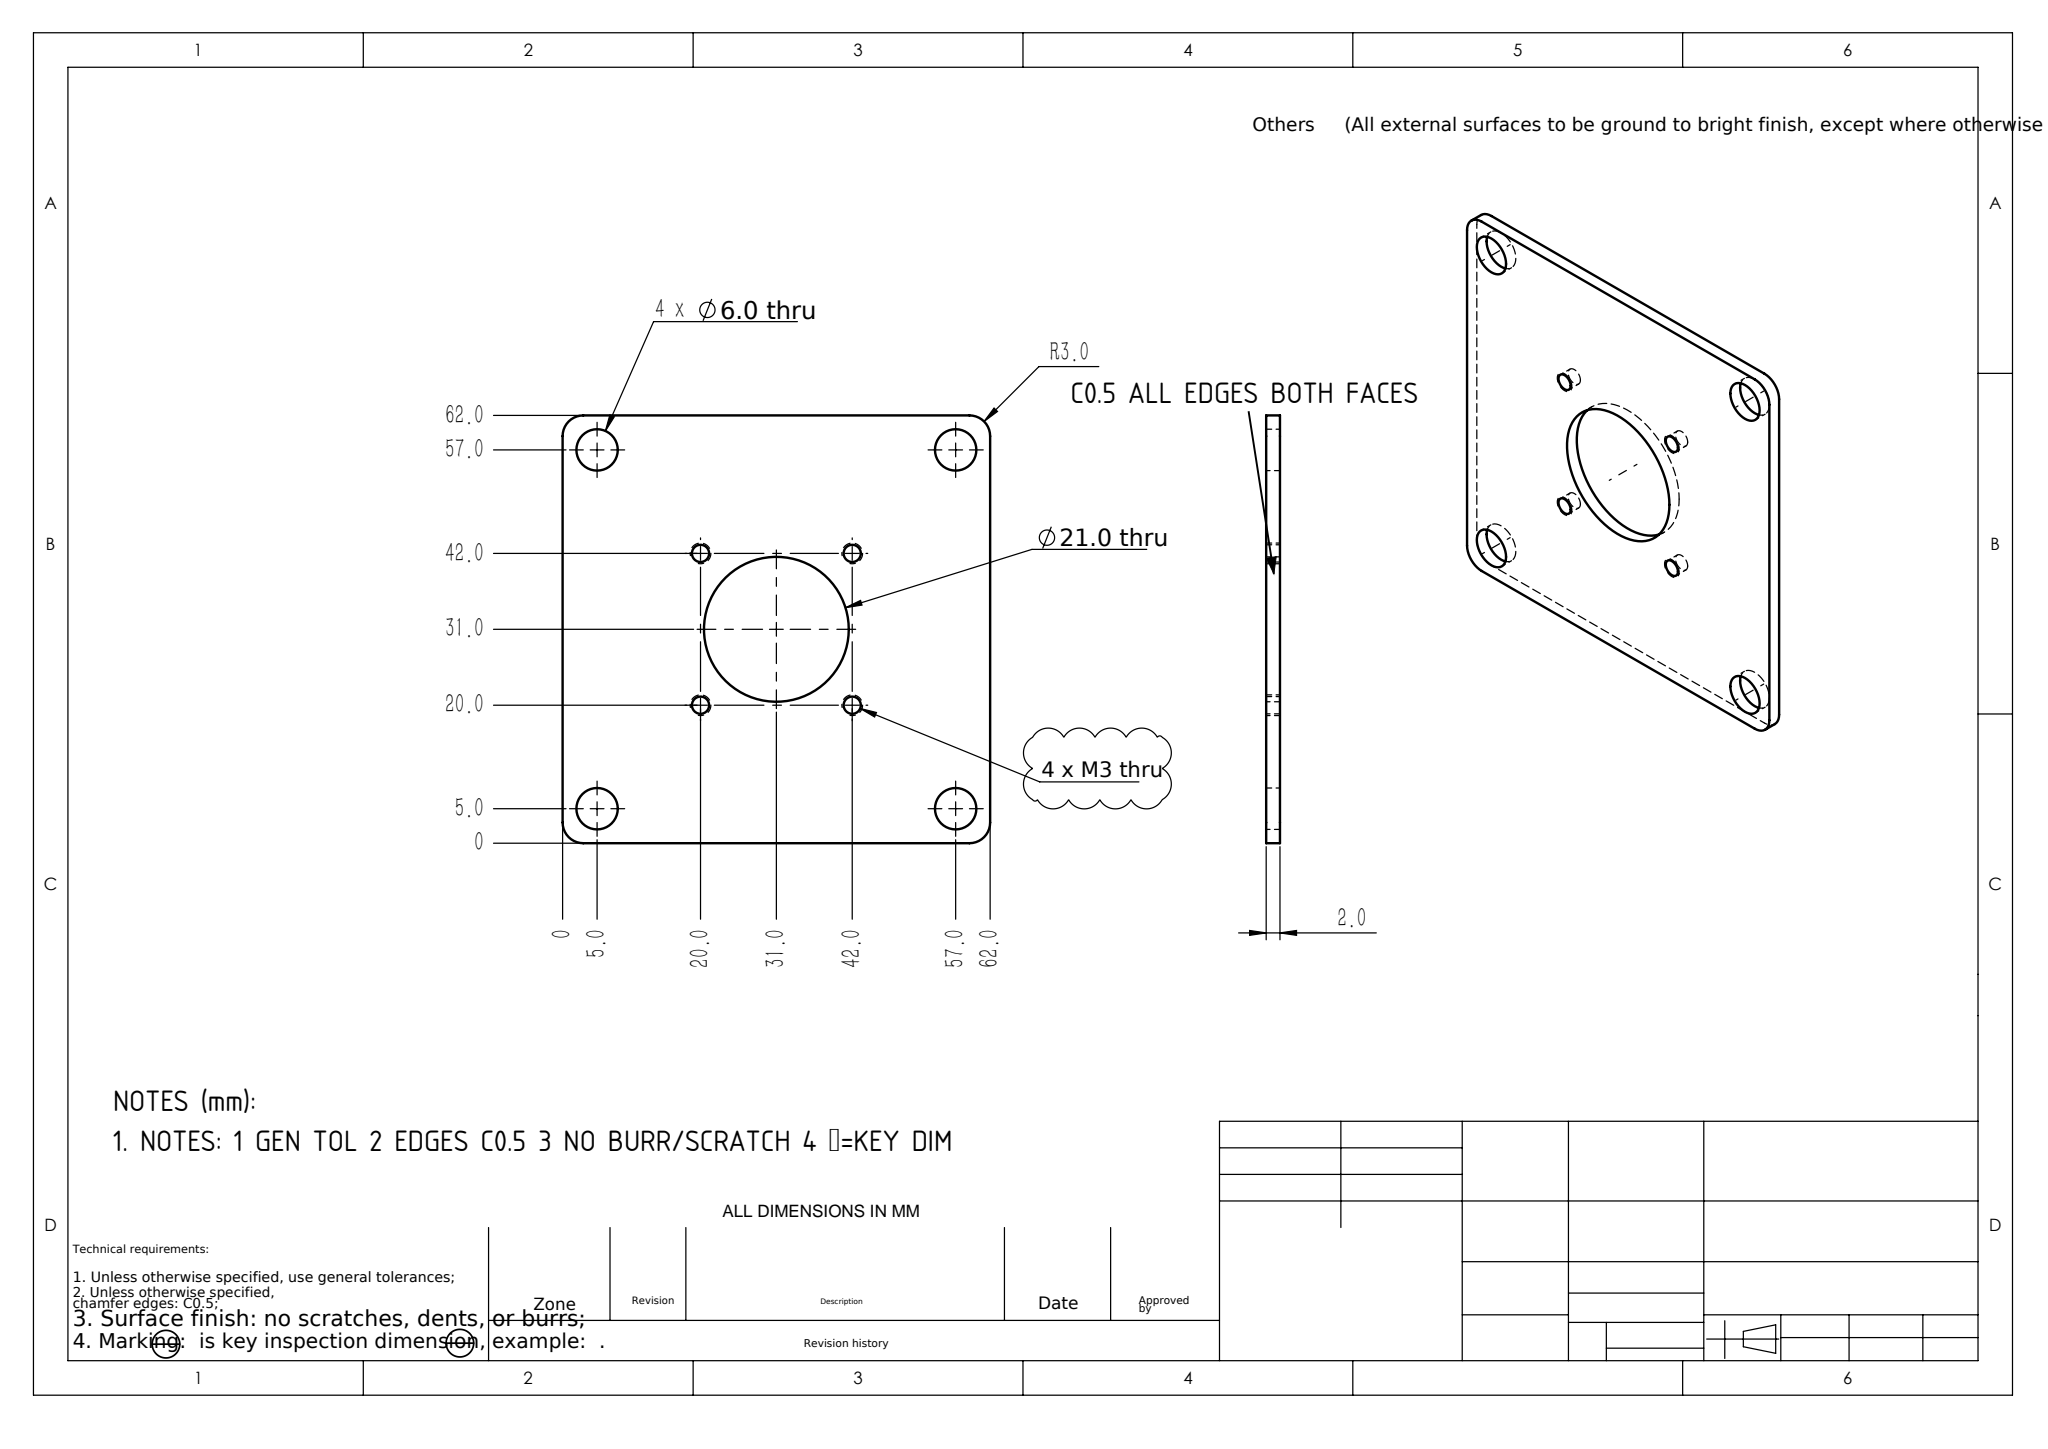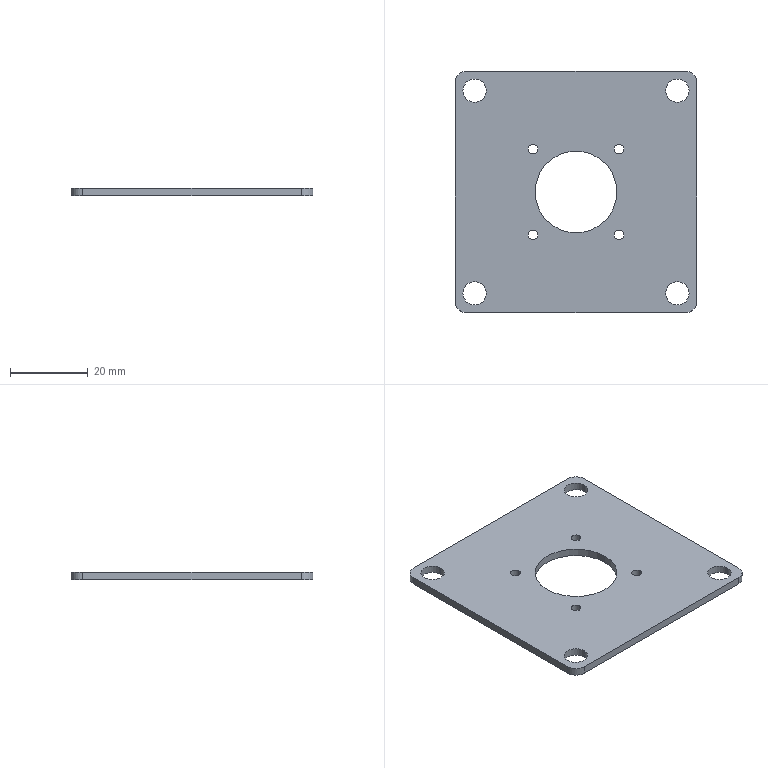Part | SolidWorks | mm | 1 solid | 28 faces | box 62 x 62 x 2 mm | volume 6714 mm3 | cylinder 22 | plane 6 | commonest cylinder face diameters 6 x12 2.5 x8 21 x2
Drawing notes:
UNLESS NOTED: BREAK ALL SHARP EDGES C0.5 (2.0 THK PLATE, BOTH FACES) | from the solid: Planes z=0.0 and z=2.0 (2.0 thk plate) with x=0/62, y=0/62 side faces; no fillet_radii or cones in STEP, so C0.5 is an unmodeled edge break
NOTES: 1 GEN TOL 2 EDGES C0.5 3 NO BURR/SCRATCH 4 Ⓒ=KEY DIM | from the solid: STEP shows plain 62.0 x 62.0 x 2.0 plate, no tol features, fillet_radii empty, cones empty: notes are general shop requirements only
build123d program:
from build123d import *

# Parameters (mm, degrees)
SKETCH1_W               = 62
SKETCH1_H               = 62
BOSS_EXTRUDE1_DEPTH     = 2
FILLET1_R               = 3
SKETCH2_R               = 10.5
CUT_EXTRUDE1_DEPTH      = 44.886
SKETCH3_R               = 3
CUT_EXTRUDE2_DEPTH      = 2
MIRROR2_COPY_1_SKETCH_R = 3
MIRROR2_COPY_1_DEPTH    = 2
M3_TAPPED_HOLE1_D       = 2.5


with BuildPart() as part:
    # Sketch1 → Boss-Extrude1 (new body)
    with BuildSketch(Plane.XY):
        Rectangle(SKETCH1_W, SKETCH1_H)
    extrude(amount=BOSS_EXTRUDE1_DEPTH)

    # Fillet1
    fillet1_edges = [part.edges().sort_by_distance(p)[0] for p in [
        (31, -31, 1),
        (-31, -31, 1),
        (-31, 31, 1),
        (31, 31, 1),
    ]]
    fillet(fillet1_edges, radius=FILLET1_R)

    # Sketch2 → Cut-Extrude1 (cut, through all)
    with BuildSketch(Plane.XY.offset(2)):
        Circle(SKETCH2_R)
    extrude(amount=-CUT_EXTRUDE1_DEPTH, mode=Mode.SUBTRACT)

    # Sketch3 → Cut-Extrude2 (cut)
    with BuildSketch(Plane.XY.offset(2)):
        with Locations((-26, 26)):
            Circle(SKETCH3_R)
    cut_extrude2 = extrude(amount=-CUT_EXTRUDE2_DEPTH, mode=Mode.SUBTRACT)

    # Mirror1: Cut-Extrude2 across plane
    add(cut_extrude2.mirror(Plane.ZX), mode=Mode.SUBTRACT)

    # Mirror2: Cut-Extrude2 across plane
    add(cut_extrude2.mirror(Plane(origin=(0, 0, 0), x_dir=(0, 0, 1), z_dir=(1, 0, 0))), mode=Mode.SUBTRACT)

    # Mirror2 copy 1 sketch → Mirror2 copy 1 (cut)
    with BuildSketch(Plane(origin=(0, 0, 2), x_dir=(-1, 0, 0), z_dir=(0, 0, 1))):
        with Locations((-26, 26)):
            Circle(MIRROR2_COPY_1_SKETCH_R)
    extrude(amount=-MIRROR2_COPY_1_DEPTH, mode=Mode.SUBTRACT)

    # M3 Tapped Hole1 (through all)
    with Locations(Plane.XY.offset(2)):
        with Locations((-11, 11), (11, 11), (11, -11), (-11, -11)):
            Hole(M3_TAPPED_HOLE1_D / 2)


solid = part.part
STEP:
#1=CARTESIAN_POINT('',(-12.25,11.,0.));
#2=VERTEX_POINT('',#1);
#3=CARTESIAN_POINT('',(-9.75,11.,0.));
#4=VERTEX_POINT('',#3);
#5=CARTESIAN_POINT('',(-11.,11.,0.));
#6=DIRECTION('',(0.,0.,1.));
#7=DIRECTION('',(1.,0.,0.));
#8=AXIS2_PLACEMENT_3D('',#5,#6,#7);
#9=CIRCLE('',#8,1.25);
#10=EDGE_CURVE('',#2,#4,#9,.T.);
#11=ORIENTED_EDGE('',*,*,#10,.F.);
#12=CARTESIAN_POINT('',(-12.25,11.,2.));
#13=VERTEX_POINT('',#12);
#14=CARTESIAN_POINT('',(-12.25,11.,2.));
#15=DIRECTION('',(0.,0.,1.));
#16=VECTOR('',#15,1000.);
#17=LINE('',#14,#16);
#18=EDGE_CURVE('',#2,#13,#17,.T.);
#19=ORIENTED_EDGE('',*,*,#18,.T.);
#20=CARTESIAN_POINT('',(-9.75,11.,2.));
#21=VERTEX_POINT('',#20);
#22=CARTESIAN_POINT('',(-11.,11.,2.));
#23=DIRECTION('',(0.,0.,1.));
#24=DIRECTION('',(1.,0.,0.));
#25=AXIS2_PLACEMENT_3D('',#22,#23,#24);
#26=CIRCLE('',#25,1.25);
#27=EDGE_CURVE('',#13,#21,#26,.T.);
#28=ORIENTED_EDGE('',*,*,#27,.T.);
#29=CARTESIAN_POINT('',(-9.75,11.,2.));
#30=DIRECTION('',(0.,0.,1.));
#31=VECTOR('',#30,1000.);
#32=LINE('',#29,#31);
#33=EDGE_CURVE('',#4,#21,#32,.T.);
#34=ORIENTED_EDGE('',*,*,#33,.F.);
#35=EDGE_LOOP('',(#11,#19,#28,#34));
#36=FACE_OUTER_BOUND('',#35,.T.);
#37=CARTESIAN_POINT('',(-11.,11.,2.));
#38=DIRECTION('',(0.,0.,1.));
#39=DIRECTION('',(1.,0.,0.));
#40=AXIS2_PLACEMENT_3D('',#37,#38,#39);
#41=CYLINDRICAL_SURFACE('',#40,1.25);
#42=ADVANCED_FACE('',(#36),#41,.F.);
#43=CARTESIAN_POINT('',(9.75,11.,0.));
#44=VERTEX_POINT('',#43);
#45=CARTESIAN_POINT('',(12.25,11.,0.));
#46=VERTEX_POINT('',#45);
#47=CARTESIAN_POINT('',(11.,11.,0.));
#48=DIRECTION('',(0.,0.,1.));
#49=DIRECTION('',(1.,0.,0.));
#50=AXIS2_PLACEMENT_3D('',#47,#48,#49);
#51=CIRCLE('',#50,1.25);
#52=EDGE_CURVE('',#44,#46,#51,.T.);
#53=ORIENTED_EDGE('',*,*,#52,.F.);
#54=CARTESIAN_POINT('',(9.75,11.,2.));
#55=VERTEX_POINT('',#54);
#56=CARTESIAN_POINT('',(9.75,11.,2.));
#57=DIRECTION('',(0.,0.,1.));
#58=VECTOR('',#57,1000.);
#59=LINE('',#56,#58);
#60=EDGE_CURVE('',#44,#55,#59,.T.);
#61=ORIENTED_EDGE('',*,*,#60,.T.);
#62=CARTESIAN_POINT('',(12.25,11.,2.));
#63=VERTEX_POINT('',#62);
#64=CARTESIAN_POINT('',(11.,11.,2.));
#65=DIRECTION('',(0.,0.,1.));
#66=DIRECTION('',(1.,0.,0.));
#67=AXIS2_PLACEMENT_3D('',#64,#65,#66);
#68=CIRCLE('',#67,1.25);
#69=EDGE_CURVE('',#55,#63,#68,.T.);
#70=ORIENTED_EDGE('',*,*,#69,.T.);
#71=CARTESIAN_POINT('',(12.25,11.,2.));
#72=DIRECTION('',(0.,0.,1.));
#73=VECTOR('',#72,1000.);
#74=LINE('',#71,#73);
#75=EDGE_CURVE('',#46,#63,#74,.T.);
#76=ORIENTED_EDGE('',*,*,#75,.F.);
#77=EDGE_LOOP('',(#53,#61,#70,#76));
#78=FACE_OUTER_BOUND('',#77,.T.);
#79=CARTESIAN_POINT('',(11.,11.,2.));
#80=DIRECTION('',(0.,0.,1.));
#81=DIRECTION('',(1.,0.,0.));
#82=AXIS2_PLACEMENT_3D('',#79,#80,#81);
#83=CYLINDRICAL_SURFACE('',#82,1.25);
#84=ADVANCED_FACE('',(#78),#83,.F.);
#85=CARTESIAN_POINT('',(9.75,-11.,0.));
#86=VERTEX_POINT('',#85);
#87=CARTESIAN_POINT('',(12.25,-11.,0.));
#88=VERTEX_POINT('',#87);
#89=CARTESIAN_POINT('',(11.,-11.,0.));
#90=DIRECTION('',(0.,0.,1.));
#91=DIRECTION('',(1.,0.,0.));
#92=AXIS2_PLACEMENT_3D('',#89,#90,#91);
#93=CIRCLE('',#92,1.25);
#94=EDGE_CURVE('',#86,#88,#93,.T.);
#95=ORIENTED_EDGE('',*,*,#94,.F.);
#96=CARTESIAN_POINT('',(9.75,-11.,2.));
#97=VERTEX_POINT('',#96);
#98=CARTESIAN_POINT('',(9.75,-11.,2.));
#99=DIRECTION('',(0.,0.,1.));
#100=VECTOR('',#99,1000.);
#101=LINE('',#98,#100);
#102=EDGE_CURVE('',#86,#97,#101,.T.);
#103=ORIENTED_EDGE('',*,*,#102,.T.);
#104=CARTESIAN_POINT('',(12.25,-11.,2.));
#105=VERTEX_POINT('',#104);
#106=CARTESIAN_POINT('',(11.,-11.,2.));
#107=DIRECTION('',(0.,0.,1.));
#108=DIRECTION('',(1.,0.,0.));
#109=AXIS2_PLACEMENT_3D('',#106,#107,#108);
#110=CIRCLE('',#109,1.25);
#111=EDGE_CURVE('',#97,#105,#110,.T.);
#112=ORIENTED_EDGE('',*,*,#111,.T.);
#113=CARTESIAN_POINT('',(12.25,-11.,2.));
#114=DIRECTION('',(0.,0.,1.));
#115=VECTOR('',#114,1000.);
#116=LINE('',#113,#115);
#117=EDGE_CURVE('',#88,#105,#116,.T.);
#118=ORIENTED_EDGE('',*,*,#117,.F.);
#119=EDGE_LOOP('',(#95,#103,#112,#118));
#120=FACE_OUTER_BOUND('',#119,.T.);
#121=CARTESIAN_POINT('',(11.,-11.,2.));
#122=DIRECTION('',(0.,0.,1.));
#123=DIRECTION('',(1.,0.,0.));
#124=AXIS2_PLACEMENT_3D('',#121,#122,#123);
#125=CYLINDRICAL_SURFACE('',#124,1.25);
#126=ADVANCED_FACE('',(#120),#125,.F.);
#127=CARTESIAN_POINT('',(-12.25,-11.,0.));
#128=VERTEX_POINT('',#127);
#129=CARTESIAN_POINT('',(-9.75,-11.,0.));
#130=VERTEX_POINT('',#129);
#131=CARTESIAN_POINT('',(-11.,-11.,0.));
#132=DIRECTION('',(0.,0.,1.));
#133=DIRECTION('',(1.,0.,0.));
#134=AXIS2_PLACEMENT_3D('',#131,#132,#133);
#135=CIRCLE('',#134,1.25);
#136=EDGE_CURVE('',#128,#130,#135,.T.);
#137=ORIENTED_EDGE('',*,*,#136,.F.);
#138=CARTESIAN_POINT('',(-12.25,-11.,2.));
#139=VERTEX_POINT('',#138);
#140=CARTESIAN_POINT('',(-12.25,-11.,2.));
#141=DIRECTION('',(0.,0.,1.));
#142=VECTOR('',#141,1000.);
#143=LINE('',#140,#142);
#144=EDGE_CURVE('',#128,#139,#143,.T.);
#145=ORIENTED_EDGE('',*,*,#144,.T.);
#146=CARTESIAN_POINT('',(-9.75,-11.,2.));
#147=VERTEX_POINT('',#146);
#148=CARTESIAN_POINT('',(-11.,-11.,2.));
#149=DIRECTION('',(0.,0.,1.));
#150=DIRECTION('',(1.,0.,0.));
#151=AXIS2_PLACEMENT_3D('',#148,#149,#150);
#152=CIRCLE('',#151,1.25);
#153=EDGE_CURVE('',#139,#147,#152,.T.);
#154=ORIENTED_EDGE('',*,*,#153,.T.);
#155=CARTESIAN_POINT('',(-9.75,-11.,2.));
#156=DIRECTION('',(0.,0.,1.));
#157=VECTOR('',#156,1000.);
#158=LINE('',#155,#157);
#159=EDGE_CURVE('',#130,#147,#158,.T.);
#160=ORIENTED_EDGE('',*,*,#159,.F.);
#161=EDGE_LOOP('',(#137,#145,#154,#160));
#162=FACE_OUTER_BOUND('',#161,.T.);
#163=CARTESIAN_POINT('',(-11.,-11.,2.));
#164=DIRECTION('',(0.,0.,1.));
#165=DIRECTION('',(1.,0.,0.));
#166=AXIS2_PLACEMENT_3D('',#163,#164,#165);
#167=CYLINDRICAL_SURFACE('',#166,1.25);
#168=ADVANCED_FACE('',(#162),#167,.F.);
#169=CARTESIAN_POINT('',(29.,26.,0.));
#170=VERTEX_POINT('',#169);
#171=CARTESIAN_POINT('',(23.,26.,0.));
#172=VERTEX_POINT('',#171);
#173=CARTESIAN_POINT('',(26.,26.,0.));
#174=DIRECTION('',(0.,0.,-1.));
#175=DIRECTION('',(-1.,0.,0.));
#176=AXIS2_PLACEMENT_3D('',#173,#174,#175);
#177=CIRCLE('',#176,3.);
#178=EDGE_CURVE('',#170,#172,#177,.T.);
#179=ORIENTED_EDGE('',*,*,#178,.T.);
#180=CARTESIAN_POINT('',(23.,26.,2.));
#181=VERTEX_POINT('',#180);
#182=CARTESIAN_POINT('',(23.,26.,-8.485));
#183=DIRECTION('',(0.,0.,1.));
#184=VECTOR('',#183,1000.);
#185=LINE('',#182,#184);
#186=EDGE_CURVE('',#172,#181,#185,.T.);
#187=ORIENTED_EDGE('',*,*,#186,.T.);
#188=CARTESIAN_POINT('',(29.,26.,2.));
#189=VERTEX_POINT('',#188);
#190=CARTESIAN_POINT('',(26.,26.,2.));
#191=DIRECTION('',(0.,0.,-1.));
#192=DIRECTION('',(-1.,0.,0.));
#193=AXIS2_PLACEMENT_3D('',#190,#191,#192);
#194=CIRCLE('',#193,3.);
#195=EDGE_CURVE('',#189,#181,#194,.T.);
#196=ORIENTED_EDGE('',*,*,#195,.F.);
#197=CARTESIAN_POINT('',(29.,26.,-8.485));
#198=DIRECTION('',(0.,0.,1.));
#199=VECTOR('',#198,1000.);
#200=LINE('',#197,#199);
#201=EDGE_CURVE('',#170,#189,#200,.T.);
#202=ORIENTED_EDGE('',*,*,#201,.F.);
#203=EDGE_LOOP('',(#179,#187,#196,#202));
#204=FACE_OUTER_BOUND('',#203,.T.);
#205=CARTESIAN_POINT('',(26.,26.,-8.485));
#206=DIRECTION('',(0.,0.,1.));
#207=DIRECTION('',(1.,0.,0.));
#208=AXIS2_PLACEMENT_3D('',#205,#206,#207);
#209=CYLINDRICAL_SURFACE('',#208,3.);
#210=ADVANCED_FACE('',(#204),#209,.F.);
#211=CARTESIAN_POINT('',(23.,-26.,0.));
#212=VERTEX_POINT('',#211);
#213=CARTESIAN_POINT('',(29.,-26.,0.));
#214=VERTEX_POINT('',#213);
#215=CARTESIAN_POINT('',(26.,-26.,0.));
#216=DIRECTION('',(0.,0.,1.));
#217=DIRECTION('',(-1.,0.,0.));
#218=AXIS2_PLACEMENT_3D('',#215,#216,#217);
#219=CIRCLE('',#218,3.);
#220=EDGE_CURVE('',#212,#214,#219,.T.);
#221=ORIENTED_EDGE('',*,*,#220,.F.);
#222=CARTESIAN_POINT('',(23.,-26.,2.));
#223=VERTEX_POINT('',#222);
#224=CARTESIAN_POINT('',(23.,-26.,-8.485));
#225=DIRECTION('',(0.,0.,1.));
#226=VECTOR('',#225,1000.);
#227=LINE('',#224,#226);
#228=EDGE_CURVE('',#212,#223,#227,.T.);
#229=ORIENTED_EDGE('',*,*,#228,.T.);
#230=CARTESIAN_POINT('',(29.,-26.,2.));
#231=VERTEX_POINT('',#230);
#232=CARTESIAN_POINT('',(26.,-26.,2.));
#233=DIRECTION('',(0.,0.,1.));
#234=DIRECTION('',(-1.,0.,0.));
#235=AXIS2_PLACEMENT_3D('',#232,#233,#234);
#236=CIRCLE('',#235,3.);
#237=EDGE_CURVE('',#223,#231,#236,.T.);
#238=ORIENTED_EDGE('',*,*,#237,.T.);
#239=CARTESIAN_POINT('',(29.,-26.,-8.485));
#240=DIRECTION('',(0.,0.,1.));
#241=VECTOR('',#240,1000.);
#242=LINE('',#239,#241);
#243=EDGE_CURVE('',#214,#231,#242,.T.);
#244=ORIENTED_EDGE('',*,*,#243,.F.);
#245=EDGE_LOOP('',(#221,#229,#238,#244));
#246=FACE_OUTER_BOUND('',#245,.T.);
#247=CARTESIAN_POINT('',(26.,-26.,-8.485));
#248=DIRECTION('',(0.,0.,1.));
#249=DIRECTION('',(1.,0.,0.));
#250=AXIS2_PLACEMENT_3D('',#247,#248,#249);
#251=CYLINDRICAL_SURFACE('',#250,3.);
#252=ADVANCED_FACE('',(#246),#251,.F.);
#253=CARTESIAN_POINT('',(-23.,-26.,0.));
#254=VERTEX_POINT('',#253);
#255=CARTESIAN_POINT('',(-29.,-26.,0.));
#256=VERTEX_POINT('',#255);
#257=CARTESIAN_POINT('',(-26.,-26.,0.));
#258=DIRECTION('',(0.,0.,-1.));
#259=DIRECTION('',(-1.,0.,0.));
#260=AXIS2_PLACEMENT_3D('',#257,#258,#259);
#261=CIRCLE('',#260,3.);
#262=EDGE_CURVE('',#254,#256,#261,.T.);
#263=ORIENTED_EDGE('',*,*,#262,.T.);
#264=CARTESIAN_POINT('',(-29.,-26.,2.));
#265=VERTEX_POINT('',#264);
#266=CARTESIAN_POINT('',(-29.,-26.,-8.485));
#267=DIRECTION('',(0.,0.,1.));
#268=VECTOR('',#267,1000.);
#269=LINE('',#266,#268);
#270=EDGE_CURVE('',#256,#265,#269,.T.);
#271=ORIENTED_EDGE('',*,*,#270,.T.);
#272=CARTESIAN_POINT('',(-23.,-26.,2.));
#273=VERTEX_POINT('',#272);
#274=CARTESIAN_POINT('',(-26.,-26.,2.));
#275=DIRECTION('',(0.,0.,-1.));
#276=DIRECTION('',(1.,0.,0.));
#277=AXIS2_PLACEMENT_3D('',#274,#275,#276);
#278=CIRCLE('',#277,3.);
#279=EDGE_CURVE('',#273,#265,#278,.T.);
#280=ORIENTED_EDGE('',*,*,#279,.F.);
#281=CARTESIAN_POINT('',(-23.,-26.,-8.485));
#282=DIRECTION('',(0.,0.,1.));
#283=VECTOR('',#282,1000.);
#284=LINE('',#281,#283);
#285=EDGE_CURVE('',#254,#273,#284,.T.);
#286=ORIENTED_EDGE('',*,*,#285,.F.);
#287=EDGE_LOOP('',(#263,#271,#280,#286));
#288=FACE_OUTER_BOUND('',#287,.T.);
#289=CARTESIAN_POINT('',(-26.,-26.,-8.485));
#290=DIRECTION('',(0.,0.,1.));
#291=DIRECTION('',(1.,0.,0.));
#292=AXIS2_PLACEMENT_3D('',#289,#290,#291);
#293=CYLINDRICAL_SURFACE('',#292,3.);
#294=ADVANCED_FACE('',(#288),#293,.F.);
#295=CARTESIAN_POINT('',(-29.,26.,0.));
#296=VERTEX_POINT('',#295);
#297=CARTESIAN_POINT('',(-23.,26.,0.));
#298=VERTEX_POINT('',#297);
#299=CARTESIAN_POINT('',(-26.,26.,0.));
#300=DIRECTION('',(0.,0.,1.));
#301=DIRECTION('',(-1.,0.,0.));
#302=AXIS2_PLACEMENT_3D('',#299,#300,#301);
#303=CIRCLE('',#302,3.);
#304=EDGE_CURVE('',#296,#298,#303,.T.);
#305=ORIENTED_EDGE('',*,*,#304,.F.);
#306=CARTESIAN_POINT('',(-29.,26.,2.));
#307=VERTEX_POINT('',#306);
#308=CARTESIAN_POINT('',(-29.,26.,-8.485));
#309=DIRECTION('',(0.,0.,1.));
#310=VECTOR('',#309,1000.);
#311=LINE('',#308,#310);
#312=EDGE_CURVE('',#296,#307,#311,.T.);
#313=ORIENTED_EDGE('',*,*,#312,.T.);
#314=CARTESIAN_POINT('',(-23.,26.,2.));
#315=VERTEX_POINT('',#314);
#316=CARTESIAN_POINT('',(-26.,26.,2.));
#317=DIRECTION('',(0.,0.,1.));
#318=DIRECTION('',(1.,0.,0.));
#319=AXIS2_PLACEMENT_3D('',#316,#317,#318);
#320=CIRCLE('',#319,3.);
#321=EDGE_CURVE('',#307,#315,#320,.T.);
#322=ORIENTED_EDGE('',*,*,#321,.T.);
#323=CARTESIAN_POINT('',(-23.,26.,-8.485));
#324=DIRECTION('',(0.,0.,1.));
#325=VECTOR('',#324,1000.);
#326=LINE('',#323,#325);
#327=EDGE_CURVE('',#298,#315,#326,.T.);
#328=ORIENTED_EDGE('',*,*,#327,.F.);
#329=EDGE_LOOP('',(#305,#313,#322,#328));
#330=FACE_OUTER_BOUND('',#329,.T.);
#331=CARTESIAN_POINT('',(-26.,26.,-8.485));
#332=DIRECTION('',(0.,0.,1.));
#333=DIRECTION('',(1.,0.,0.));
#334=AXIS2_PLACEMENT_3D('',#331,#332,#333);
#335=CYLINDRICAL_SURFACE('',#334,3.);
#336=ADVANCED_FACE('',(#330),#335,.F.);
#337=CARTESIAN_POINT('',(-10.5,0.,0.));
#338=VERTEX_POINT('',#337);
#339=CARTESIAN_POINT('',(10.5,0.,0.));
#340=VERTEX_POINT('',#339);
#341=CARTESIAN_POINT('',(0.,0.,0.));
#342=DIRECTION('',(0.,0.,1.));
#343=DIRECTION('',(1.,0.,0.));
#344=AXIS2_PLACEMENT_3D('',#341,#342,#343);
#345=CIRCLE('',#344,10.5);
#346=EDGE_CURVE('',#338,#340,#345,.T.);
#347=ORIENTED_EDGE('',*,*,#346,.F.);
#348=CARTESIAN_POINT('',(-10.5,0.,2.));
#349=VERTEX_POINT('',#348);
#350=CARTESIAN_POINT('',(-10.5,0.,0.));
#351=DIRECTION('',(0.,0.,1.));
#352=VECTOR('',#351,1000.);
#353=LINE('',#350,#352);
#354=EDGE_CURVE('',#338,#349,#353,.T.);
#355=ORIENTED_EDGE('',*,*,#354,.T.);
#356=CARTESIAN_POINT('',(10.5,0.,2.));
#357=VERTEX_POINT('',#356);
#358=CARTESIAN_POINT('',(0.,0.,2.));
#359=DIRECTION('',(0.,0.,1.));
#360=DIRECTION('',(1.,0.,0.));
#361=AXIS2_PLACEMENT_3D('',#358,#359,#360);
#362=CIRCLE('',#361,10.5);
#363=EDGE_CURVE('',#349,#357,#362,.T.);
#364=ORIENTED_EDGE('',*,*,#363,.T.);
#365=CARTESIAN_POINT('',(10.5,0.,0.));
#366=DIRECTION('',(0.,0.,1.));
#367=VECTOR('',#366,1000.);
#368=LINE('',#365,#367);
#369=EDGE_CURVE('',#340,#357,#368,.T.);
#370=ORIENTED_EDGE('',*,*,#369,.F.);
#371=EDGE_LOOP('',(#347,#355,#364,#370));
#372=FACE_OUTER_BOUND('',#371,.T.);
#373=CARTESIAN_POINT('',(0.,0.,0.));
#374=DIRECTION('',(0.,0.,1.));
#375=DIRECTION('',(1.,0.,0.));
#376=AXIS2_PLACEMENT_3D('',#373,#374,#375);
#377=CYLINDRICAL_SURFACE('',#376,10.5);
#378=ADVANCED_FACE('',(#372),#377,.F.);
#379=CARTESIAN_POINT('',(-11.,11.,0.));
#380=DIRECTION('',(0.,0.,1.));
#381=DIRECTION('',(1.,0.,0.));
#382=AXIS2_PLACEMENT_3D('',#379,#380,#381);
#383=CIRCLE('',#382,1.25);
#384=EDGE_CURVE('',#4,#2,#383,.T.);
#385=ORIENTED_EDGE('',*,*,#384,.T.);
#386=ORIENTED_EDGE('',*,*,#10,.T.);
#387=EDGE_LOOP('',(#385,#386));
#388=FACE_BOUND('',#387,.T.);
#389=CARTESIAN_POINT('',(11.,11.,0.));
#390=DIRECTION('',(0.,0.,1.));
#391=DIRECTION('',(1.,0.,0.));
#392=AXIS2_PLACEMENT_3D('',#389,#390,#391);
#393=CIRCLE('',#392,1.25);
#394=EDGE_CURVE('',#46,#44,#393,.T.);
#395=ORIENTED_EDGE('',*,*,#394,.T.);
#396=ORIENTED_EDGE('',*,*,#52,.T.);
#397=EDGE_LOOP('',(#395,#396));
#398=FACE_BOUND('',#397,.T.);
#399=CARTESIAN_POINT('',(11.,-11.,0.));
#400=DIRECTION('',(0.,0.,1.));
#401=DIRECTION('',(1.,0.,0.));
#402=AXIS2_PLACEMENT_3D('',#399,#400,#401);
#403=CIRCLE('',#402,1.25);
#404=EDGE_CURVE('',#88,#86,#403,.T.);
#405=ORIENTED_EDGE('',*,*,#404,.T.);
#406=ORIENTED_EDGE('',*,*,#94,.T.);
#407=EDGE_LOOP('',(#405,#406));
#408=FACE_BOUND('',#407,.T.);
#409=CARTESIAN_POINT('',(31.,-28.,0.));
#410=VERTEX_POINT('',#409);
#411=CARTESIAN_POINT('',(31.,28.,0.));
#412=VERTEX_POINT('',#411);
#413=CARTESIAN_POINT('',(31.,-31.,0.));
#414=DIRECTION('',(0.,1.,0.));
#415=VECTOR('',#414,1000.);
#416=LINE('',#413,#415);
#417=EDGE_CURVE('',#410,#412,#416,.T.);
#418=ORIENTED_EDGE('',*,*,#417,.F.);
#419=CARTESIAN_POINT('',(28.,-31.,0.));
#420=VERTEX_POINT('',#419);
#421=CARTESIAN_POINT('',(28.,-28.,0.));
#422=DIRECTION('',(0.,0.,-1.));
#423=DIRECTION('',(-1.,0.,0.));
#424=AXIS2_PLACEMENT_3D('',#421,#422,#423);
#425=CIRCLE('',#424,3.);
#426=EDGE_CURVE('',#410,#420,#425,.T.);
#427=ORIENTED_EDGE('',*,*,#426,.T.);
#428=CARTESIAN_POINT('',(-28.,-31.,0.));
#429=VERTEX_POINT('',#428);
#430=CARTESIAN_POINT('',(-31.,-31.,0.));
#431=DIRECTION('',(1.,0.,0.));
#432=VECTOR('',#431,1000.);
#433=LINE('',#430,#432);
#434=EDGE_CURVE('',#429,#420,#433,.T.);
#435=ORIENTED_EDGE('',*,*,#434,.F.);
#436=CARTESIAN_POINT('',(-31.,-28.,0.));
#437=VERTEX_POINT('',#436);
#438=CARTESIAN_POINT('',(-28.,-28.,0.));
#439=DIRECTION('',(0.,0.,-1.));
#440=DIRECTION('',(-1.,0.,0.));
#441=AXIS2_PLACEMENT_3D('',#438,#439,#440);
#442=CIRCLE('',#441,3.);
#443=EDGE_CURVE('',#429,#437,#442,.T.);
#444=ORIENTED_EDGE('',*,*,#443,.T.);
#445=CARTESIAN_POINT('',(-31.,28.,0.));
#446=VERTEX_POINT('',#445);
#447=CARTESIAN_POINT('',(-31.,-31.,0.));
#448=DIRECTION('',(0.,-1.,0.));
#449=VECTOR('',#448,1000.);
#450=LINE('',#447,#449);
#451=EDGE_CURVE('',#446,#437,#450,.T.);
#452=ORIENTED_EDGE('',*,*,#451,.F.);
#453=CARTESIAN_POINT('',(-28.,31.,0.));
#454=VERTEX_POINT('',#453);
#455=CARTESIAN_POINT('',(-28.,28.,0.));
#456=DIRECTION('',(0.,0.,-1.));
#457=DIRECTION('',(-1.,0.,0.));
#458=AXIS2_PLACEMENT_3D('',#455,#456,#457);
#459=CIRCLE('',#458,3.);
#460=EDGE_CURVE('',#446,#454,#459,.T.);
#461=ORIENTED_EDGE('',*,*,#460,.T.);
#462=CARTESIAN_POINT('',(28.,31.,0.));
#463=VERTEX_POINT('',#462);
#464=CARTESIAN_POINT('',(-31.,31.,0.));
#465=DIRECTION('',(-1.,0.,0.));
#466=VECTOR('',#465,1000.);
#467=LINE('',#464,#466);
#468=EDGE_CURVE('',#463,#454,#467,.T.);
#469=ORIENTED_EDGE('',*,*,#468,.F.);
#470=CARTESIAN_POINT('',(28.,28.,0.));
#471=DIRECTION('',(0.,0.,-1.));
#472=DIRECTION('',(-1.,0.,0.));
#473=AXIS2_PLACEMENT_3D('',#470,#471,#472);
#474=CIRCLE('',#473,3.);
#475=EDGE_CURVE('',#463,#412,#474,.T.);
#476=ORIENTED_EDGE('',*,*,#475,.T.);
#477=EDGE_LOOP('',(#418,#427,#435,#444,#452,#461,#469,#476));
#478=FACE_OUTER_BOUND('',#477,.T.);
#479=CARTESIAN_POINT('',(0.,0.,0.));
#480=DIRECTION('',(0.,0.,1.));
#481=DIRECTION('',(1.,0.,0.));
#482=AXIS2_PLACEMENT_3D('',#479,#480,#481);
#483=CIRCLE('',#482,10.5);
#484=EDGE_CURVE('',#340,#338,#483,.T.);
#485=ORIENTED_EDGE('',*,*,#484,.T.);
#486=ORIENTED_EDGE('',*,*,#346,.T.);
#487=EDGE_LOOP('',(#485,#486));
#488=FACE_BOUND('',#487,.T.);
#489=CARTESIAN_POINT('',(-26.,26.,0.));
#490=DIRECTION('',(0.,0.,1.));
#491=DIRECTION('',(-1.,0.,0.));
#492=AXIS2_PLACEMENT_3D('',#489,#490,#491);
#493=CIRCLE('',#492,3.);
#494=EDGE_CURVE('',#298,#296,#493,.T.);
#495=ORIENTED_EDGE('',*,*,#494,.T.);
#496=ORIENTED_EDGE('',*,*,#304,.T.);
#497=EDGE_LOOP('',(#495,#496));
#498=FACE_BOUND('',#497,.T.);
#499=ORIENTED_EDGE('',*,*,#262,.F.);
#500=CARTESIAN_POINT('',(-26.,-26.,0.));
#501=DIRECTION('',(0.,0.,-1.));
#502=DIRECTION('',(-1.,0.,0.));
#503=AXIS2_PLACEMENT_3D('',#500,#501,#502);
#504=CIRCLE('',#503,3.);
#505=EDGE_CURVE('',#256,#254,#504,.T.);
#506=ORIENTED_EDGE('',*,*,#505,.F.);
#507=EDGE_LOOP('',(#499,#506));
#508=FACE_BOUND('',#507,.T.);
#509=CARTESIAN_POINT('',(26.,-26.,0.));
#510=DIRECTION('',(0.,0.,1.));
#511=DIRECTION('',(-1.,0.,0.));
#512=AXIS2_PLACEMENT_3D('',#509,#510,#511);
#513=CIRCLE('',#512,3.);
#514=EDGE_CURVE('',#214,#212,#513,.T.);
#515=ORIENTED_EDGE('',*,*,#514,.T.);
#516=ORIENTED_EDGE('',*,*,#220,.T.);
#517=EDGE_LOOP('',(#515,#516));
#518=FACE_BOUND('',#517,.T.);
#519=ORIENTED_EDGE('',*,*,#178,.F.);
#520=CARTESIAN_POINT('',(26.,26.,0.));
#521=DIRECTION('',(0.,0.,-1.));
#522=DIRECTION('',(-1.,0.,0.));
#523=AXIS2_PLACEMENT_3D('',#520,#521,#522);
#524=CIRCLE('',#523,3.);
#525=EDGE_CURVE('',#172,#170,#524,.T.);
#526=ORIENTED_EDGE('',*,*,#525,.F.);
#527=EDGE_LOOP('',(#519,#526));
#528=FACE_BOUND('',#527,.T.);
#529=CARTESIAN_POINT('',(-11.,-11.,0.));
#530=DIRECTION('',(0.,0.,1.));
#531=DIRECTION('',(1.,0.,0.));
#532=AXIS2_PLACEMENT_3D('',#529,#530,#531);
#533=CIRCLE('',#532,1.25);
#534=EDGE_CURVE('',#130,#128,#533,.T.);
#535=ORIENTED_EDGE('',*,*,#534,.T.);
#536=ORIENTED_EDGE('',*,*,#136,.T.);
#537=EDGE_LOOP('',(#535,#536));
#538=FACE_BOUND('',#537,.T.);
#539=CARTESIAN_POINT('',(0.,0.,0.));
#540=DIRECTION('',(0.,0.,-1.));
#541=DIRECTION('',(-1.,0.,0.));
#542=AXIS2_PLACEMENT_3D('',#539,#540,#541);
#543=PLANE('',#542);
#544=ADVANCED_FACE('',(#388,#398,#408,#478,#488,#498,#508,#518,#528,#538),#543,.T.);
#545=CARTESIAN_POINT('',(31.,-28.,2.));
#546=VERTEX_POINT('',#545);
#547=CARTESIAN_POINT('',(31.,28.,2.));
#548=VERTEX_POINT('',#547);
#549=CARTESIAN_POINT('',(31.,-31.,2.));
#550=DIRECTION('',(0.,1.,0.));
#551=VECTOR('',#550,1000.);
#552=LINE('',#549,#551);
#553=EDGE_CURVE('',#546,#548,#552,.T.);
#554=ORIENTED_EDGE('',*,*,#553,.F.);
#555=CARTESIAN_POINT('',(31.,-28.,2.));
#556=DIRECTION('',(0.,0.,-1.));
#557=VECTOR('',#556,1000.);
#558=LINE('',#555,#557);
#559=EDGE_CURVE('',#546,#410,#558,.T.);
#560=ORIENTED_EDGE('',*,*,#559,.T.);
#561=ORIENTED_EDGE('',*,*,#417,.T.);
#562=CARTESIAN_POINT('',(31.,28.,2.));
#563=DIRECTION('',(0.,0.,1.));
#564=VECTOR('',#563,1000.);
#565=LINE('',#562,#564);
#566=EDGE_CURVE('',#412,#548,#565,.T.);
#567=ORIENTED_EDGE('',*,*,#566,.T.);
#568=EDGE_LOOP('',(#554,#560,#561,#567));
#569=FACE_OUTER_BOUND('',#568,.T.);
#570=CARTESIAN_POINT('',(31.,-31.,2.));
#571=DIRECTION('',(-1.,0.,0.));
#572=DIRECTION('',(0.,0.,1.));
#573=AXIS2_PLACEMENT_3D('',#570,#571,#572);
#574=PLANE('',#573);
#575=ADVANCED_FACE('',(#569),#574,.F.);
#576=ORIENTED_EDGE('',*,*,#468,.T.);
#577=CARTESIAN_POINT('',(-28.,31.,2.));
#578=VERTEX_POINT('',#577);
#579=CARTESIAN_POINT('',(-28.,31.,2.));
#580=DIRECTION('',(0.,0.,1.));
#581=VECTOR('',#580,1000.);
#582=LINE('',#579,#581);
#583=EDGE_CURVE('',#454,#578,#582,.T.);
#584=ORIENTED_EDGE('',*,*,#583,.T.);
#585=CARTESIAN_POINT('',(28.,31.,2.));
#586=VERTEX_POINT('',#585);
#587=CARTESIAN_POINT('',(-31.,31.,2.));
#588=DIRECTION('',(-1.,0.,0.));
#589=VECTOR('',#588,1000.);
#590=LINE('',#587,#589);
#591=EDGE_CURVE('',#586,#578,#590,.T.);
#592=ORIENTED_EDGE('',*,*,#591,.F.);
#593=CARTESIAN_POINT('',(28.,31.,2.));
#594=DIRECTION('',(0.,0.,-1.));
#595=VECTOR('',#594,1000.);
#596=LINE('',#593,#595);
#597=EDGE_CURVE('',#586,#463,#596,.T.);
#598=ORIENTED_EDGE('',*,*,#597,.T.);
#599=EDGE_LOOP('',(#576,#584,#592,#598));
#600=FACE_OUTER_BOUND('',#599,.T.);
#601=CARTESIAN_POINT('',(-31.,31.,2.));
#602=DIRECTION('',(0.,-1.,0.));
#603=DIRECTION('',(0.,0.,-1.));
#604=AXIS2_PLACEMENT_3D('',#601,#602,#603);
#605=PLANE('',#604);
#606=ADVANCED_FACE('',(#600),#605,.F.);
#607=ORIENTED_EDGE('',*,*,#451,.T.);
#608=CARTESIAN_POINT('',(-31.,-28.,2.));
#609=VERTEX_POINT('',#608);
#610=CARTESIAN_POINT('',(-31.,-28.,2.));
#611=DIRECTION('',(0.,0.,1.));
#612=VECTOR('',#611,1000.);
#613=LINE('',#610,#612);
#614=EDGE_CURVE('',#437,#609,#613,.T.);
#615=ORIENTED_EDGE('',*,*,#614,.T.);
#616=CARTESIAN_POINT('',(-31.,28.,2.));
#617=VERTEX_POINT('',#616);
#618=CARTESIAN_POINT('',(-31.,-31.,2.));
#619=DIRECTION('',(0.,-1.,0.));
#620=VECTOR('',#619,1000.);
#621=LINE('',#618,#620);
#622=EDGE_CURVE('',#617,#609,#621,.T.);
#623=ORIENTED_EDGE('',*,*,#622,.F.);
#624=CARTESIAN_POINT('',(-31.,28.,2.));
#625=DIRECTION('',(0.,0.,-1.));
#626=VECTOR('',#625,1000.);
#627=LINE('',#624,#626);
#628=EDGE_CURVE('',#617,#446,#627,.T.);
#629=ORIENTED_EDGE('',*,*,#628,.T.);
#630=EDGE_LOOP('',(#607,#615,#623,#629));
#631=FACE_OUTER_BOUND('',#630,.T.);
#632=CARTESIAN_POINT('',(-31.,-31.,2.));
#633=DIRECTION('',(1.,0.,0.));
#634=DIRECTION('',(0.,0.,-1.));
#635=AXIS2_PLACEMENT_3D('',#632,#633,#634);
#636=PLANE('',#635);
#637=ADVANCED_FACE('',(#631),#636,.F.);
#638=ORIENTED_EDGE('',*,*,#434,.T.);
#639=CARTESIAN_POINT('',(28.,-31.,2.));
#640=VERTEX_POINT('',#639);
#641=CARTESIAN_POINT('',(28.,-31.,2.));
#642=DIRECTION('',(0.,0.,1.));
#643=VECTOR('',#642,1000.);
#644=LINE('',#641,#643);
#645=EDGE_CURVE('',#420,#640,#644,.T.);
#646=ORIENTED_EDGE('',*,*,#645,.T.);
#647=CARTESIAN_POINT('',(-28.,-31.,2.));
#648=VERTEX_POINT('',#647);
#649=CARTESIAN_POINT('',(-31.,-31.,2.));
#650=DIRECTION('',(1.,0.,0.));
#651=VECTOR('',#650,1000.);
#652=LINE('',#649,#651);
#653=EDGE_CURVE('',#648,#640,#652,.T.);
#654=ORIENTED_EDGE('',*,*,#653,.F.);
#655=CARTESIAN_POINT('',(-28.,-31.,2.));
#656=DIRECTION('',(0.,0.,-1.));
#657=VECTOR('',#656,1000.);
#658=LINE('',#655,#657);
#659=EDGE_CURVE('',#648,#429,#658,.T.);
#660=ORIENTED_EDGE('',*,*,#659,.T.);
#661=EDGE_LOOP('',(#638,#646,#654,#660));
#662=FACE_OUTER_BOUND('',#661,.T.);
#663=CARTESIAN_POINT('',(-31.,-31.,2.));
#664=DIRECTION('',(0.,1.,0.));
#665=DIRECTION('',(0.,0.,1.));
#666=AXIS2_PLACEMENT_3D('',#663,#664,#665);
#667=PLANE('',#666);
#668=ADVANCED_FACE('',(#662),#667,.F.);
#669=CARTESIAN_POINT('',(-11.,11.,2.));
#670=DIRECTION('',(0.,0.,1.));
#671=DIRECTION('',(1.,0.,0.));
#672=AXIS2_PLACEMENT_3D('',#669,#670,#671);
#673=CIRCLE('',#672,1.25);
#674=EDGE_CURVE('',#21,#13,#673,.T.);
#675=ORIENTED_EDGE('',*,*,#674,.F.);
#676=ORIENTED_EDGE('',*,*,#27,.F.);
#677=EDGE_LOOP('',(#675,#676));
#678=FACE_BOUND('',#677,.T.);
#679=CARTESIAN_POINT('',(11.,11.,2.));
#680=DIRECTION('',(0.,0.,1.));
#681=DIRECTION('',(1.,0.,0.));
#682=AXIS2_PLACEMENT_3D('',#679,#680,#681);
#683=CIRCLE('',#682,1.25);
#684=EDGE_CURVE('',#63,#55,#683,.T.);
#685=ORIENTED_EDGE('',*,*,#684,.F.);
#686=ORIENTED_EDGE('',*,*,#69,.F.);
#687=EDGE_LOOP('',(#685,#686));
#688=FACE_BOUND('',#687,.T.);
#689=CARTESIAN_POINT('',(11.,-11.,2.));
#690=DIRECTION('',(0.,0.,1.));
#691=DIRECTION('',(1.,0.,0.));
#692=AXIS2_PLACEMENT_3D('',#689,#690,#691);
#693=CIRCLE('',#692,1.25);
#694=EDGE_CURVE('',#105,#97,#693,.T.);
#695=ORIENTED_EDGE('',*,*,#694,.F.);
#696=ORIENTED_EDGE('',*,*,#111,.F.);
#697=EDGE_LOOP('',(#695,#696));
#698=FACE_BOUND('',#697,.T.);
#699=CARTESIAN_POINT('',(-11.,-11.,2.));
#700=DIRECTION('',(0.,0.,1.));
#701=DIRECTION('',(1.,0.,0.));
#702=AXIS2_PLACEMENT_3D('',#699,#700,#701);
#703=CIRCLE('',#702,1.25);
#704=EDGE_CURVE('',#147,#139,#703,.T.);
#705=ORIENTED_EDGE('',*,*,#704,.F.);
#706=ORIENTED_EDGE('',*,*,#153,.F.);
#707=EDGE_LOOP('',(#705,#706));
#708=FACE_BOUND('',#707,.T.);
#709=ORIENTED_EDGE('',*,*,#195,.T.);
#710=CARTESIAN_POINT('',(26.,26.,2.));
#711=DIRECTION('',(0.,0.,-1.));
#712=DIRECTION('',(-1.,0.,0.));
#713=AXIS2_PLACEMENT_3D('',#710,#711,#712);
#714=CIRCLE('',#713,3.);
#715=EDGE_CURVE('',#181,#189,#714,.T.);
#716=ORIENTED_EDGE('',*,*,#715,.T.);
#717=EDGE_LOOP('',(#709,#716));
#718=FACE_BOUND('',#717,.T.);
#719=CARTESIAN_POINT('',(26.,-26.,2.));
#720=DIRECTION('',(0.,0.,1.));
#721=DIRECTION('',(-1.,0.,0.));
#722=AXIS2_PLACEMENT_3D('',#719,#720,#721);
#723=CIRCLE('',#722,3.);
#724=EDGE_CURVE('',#231,#223,#723,.T.);
#725=ORIENTED_EDGE('',*,*,#724,.F.);
#726=ORIENTED_EDGE('',*,*,#237,.F.);
#727=EDGE_LOOP('',(#725,#726));
#728=FACE_BOUND('',#727,.T.);
#729=ORIENTED_EDGE('',*,*,#279,.T.);
#730=CARTESIAN_POINT('',(-26.,-26.,2.));
#731=DIRECTION('',(0.,0.,-1.));
#732=DIRECTION('',(1.,0.,0.));
#733=AXIS2_PLACEMENT_3D('',#730,#731,#732);
#734=CIRCLE('',#733,3.);
#735=EDGE_CURVE('',#265,#273,#734,.T.);
#736=ORIENTED_EDGE('',*,*,#735,.T.);
#737=EDGE_LOOP('',(#729,#736));
#738=FACE_BOUND('',#737,.T.);
#739=CARTESIAN_POINT('',(-26.,26.,2.));
#740=DIRECTION('',(0.,0.,1.));
#741=DIRECTION('',(1.,0.,0.));
#742=AXIS2_PLACEMENT_3D('',#739,#740,#741);
#743=CIRCLE('',#742,3.);
#744=EDGE_CURVE('',#315,#307,#743,.T.);
#745=ORIENTED_EDGE('',*,*,#744,.F.);
#746=ORIENTED_EDGE('',*,*,#321,.F.);
#747=EDGE_LOOP('',(#745,#746));
#748=FACE_BOUND('',#747,.T.);
#749=CARTESIAN_POINT('',(0.,0.,2.));
#750=DIRECTION('',(0.,0.,1.));
#751=DIRECTION('',(1.,0.,0.));
#752=AXIS2_PLACEMENT_3D('',#749,#750,#751);
#753=CIRCLE('',#752,10.5);
#754=EDGE_CURVE('',#357,#349,#753,.T.);
#755=ORIENTED_EDGE('',*,*,#754,.F.);
#756=ORIENTED_EDGE('',*,*,#363,.F.);
#757=EDGE_LOOP('',(#755,#756));
#758=FACE_BOUND('',#757,.T.);
#759=ORIENTED_EDGE('',*,*,#653,.T.);
#760=CARTESIAN_POINT('',(28.,-28.,2.));
#761=DIRECTION('',(0.,0.,1.));
#762=DIRECTION('',(-1.,0.,0.));
#763=AXIS2_PLACEMENT_3D('',#760,#761,#762);
#764=CIRCLE('',#763,3.);
#765=EDGE_CURVE('',#640,#546,#764,.T.);
#766=ORIENTED_EDGE('',*,*,#765,.T.);
#767=ORIENTED_EDGE('',*,*,#553,.T.);
#768=CARTESIAN_POINT('',(28.,28.,2.));
#769=DIRECTION('',(0.,0.,1.));
#770=DIRECTION('',(-1.,0.,0.));
#771=AXIS2_PLACEMENT_3D('',#768,#769,#770);
#772=CIRCLE('',#771,3.);
#773=EDGE_CURVE('',#548,#586,#772,.T.);
#774=ORIENTED_EDGE('',*,*,#773,.T.);
#775=ORIENTED_EDGE('',*,*,#591,.T.);
#776=CARTESIAN_POINT('',(-28.,28.,2.));
#777=DIRECTION('',(0.,0.,1.));
#778=DIRECTION('',(-1.,0.,0.));
#779=AXIS2_PLACEMENT_3D('',#776,#777,#778);
#780=CIRCLE('',#779,3.);
#781=EDGE_CURVE('',#578,#617,#780,.T.);
#782=ORIENTED_EDGE('',*,*,#781,.T.);
#783=ORIENTED_EDGE('',*,*,#622,.T.);
#784=CARTESIAN_POINT('',(-28.,-28.,2.));
#785=DIRECTION('',(0.,0.,1.));
#786=DIRECTION('',(-1.,0.,0.));
#787=AXIS2_PLACEMENT_3D('',#784,#785,#786);
#788=CIRCLE('',#787,3.);
#789=EDGE_CURVE('',#609,#648,#788,.T.);
#790=ORIENTED_EDGE('',*,*,#789,.T.);
#791=EDGE_LOOP('',(#759,#766,#767,#774,#775,#782,#783,#790));
#792=FACE_OUTER_BOUND('',#791,.T.);
#793=CARTESIAN_POINT('',(0.,0.,2.));
#794=DIRECTION('',(0.,0.,-1.));
#795=DIRECTION('',(-1.,0.,0.));
#796=AXIS2_PLACEMENT_3D('',#793,#794,#795);
#797=PLANE('',#796);
#798=ADVANCED_FACE('',(#678,#688,#698,#708,#718,#728,#738,#748,#758,#792),#797,.F.);
#799=ORIENTED_EDGE('',*,*,#765,.F.);
#800=ORIENTED_EDGE('',*,*,#645,.F.);
#801=ORIENTED_EDGE('',*,*,#426,.F.);
#802=ORIENTED_EDGE('',*,*,#559,.F.);
#803=EDGE_LOOP('',(#799,#800,#801,#802));
#804=FACE_OUTER_BOUND('',#803,.T.);
#805=CARTESIAN_POINT('',(28.,-28.,2.));
#806=DIRECTION('',(0.,0.,-1.));
#807=DIRECTION('',(-1.,0.,0.));
#808=AXIS2_PLACEMENT_3D('',#805,#806,#807);
#809=CYLINDRICAL_SURFACE('',#808,3.);
#810=ADVANCED_FACE('',(#804),#809,.T.);
#811=ORIENTED_EDGE('',*,*,#789,.F.);
#812=ORIENTED_EDGE('',*,*,#614,.F.);
#813=ORIENTED_EDGE('',*,*,#443,.F.);
#814=ORIENTED_EDGE('',*,*,#659,.F.);
#815=EDGE_LOOP('',(#811,#812,#813,#814));
#816=FACE_OUTER_BOUND('',#815,.T.);
#817=CARTESIAN_POINT('',(-28.,-28.,2.));
#818=DIRECTION('',(0.,0.,-1.));
#819=DIRECTION('',(-1.,0.,0.));
#820=AXIS2_PLACEMENT_3D('',#817,#818,#819);
#821=CYLINDRICAL_SURFACE('',#820,3.);
#822=ADVANCED_FACE('',(#816),#821,.T.);
#823=ORIENTED_EDGE('',*,*,#781,.F.);
#824=ORIENTED_EDGE('',*,*,#583,.F.);
#825=ORIENTED_EDGE('',*,*,#460,.F.);
#826=ORIENTED_EDGE('',*,*,#628,.F.);
#827=EDGE_LOOP('',(#823,#824,#825,#826));
#828=FACE_OUTER_BOUND('',#827,.T.);
#829=CARTESIAN_POINT('',(-28.,28.,2.));
#830=DIRECTION('',(0.,0.,-1.));
#831=DIRECTION('',(-1.,0.,0.));
#832=AXIS2_PLACEMENT_3D('',#829,#830,#831);
#833=CYLINDRICAL_SURFACE('',#832,3.);
#834=ADVANCED_FACE('',(#828),#833,.T.);
#835=ORIENTED_EDGE('',*,*,#773,.F.);
#836=ORIENTED_EDGE('',*,*,#566,.F.);
#837=ORIENTED_EDGE('',*,*,#475,.F.);
#838=ORIENTED_EDGE('',*,*,#597,.F.);
#839=EDGE_LOOP('',(#835,#836,#837,#838));
#840=FACE_OUTER_BOUND('',#839,.T.);
#841=CARTESIAN_POINT('',(28.,28.,2.));
#842=DIRECTION('',(0.,0.,-1.));
#843=DIRECTION('',(-1.,0.,0.));
#844=AXIS2_PLACEMENT_3D('',#841,#842,#843);
#845=CYLINDRICAL_SURFACE('',#844,3.);
#846=ADVANCED_FACE('',(#840),#845,.T.);
#847=ORIENTED_EDGE('',*,*,#354,.F.);
#848=ORIENTED_EDGE('',*,*,#484,.F.);
#849=ORIENTED_EDGE('',*,*,#369,.T.);
#850=ORIENTED_EDGE('',*,*,#754,.T.);
#851=EDGE_LOOP('',(#847,#848,#849,#850));
#852=FACE_OUTER_BOUND('',#851,.T.);
#853=CARTESIAN_POINT('',(0.,0.,0.));
#854=DIRECTION('',(0.,0.,1.));
#855=DIRECTION('',(1.,0.,0.));
#856=AXIS2_PLACEMENT_3D('',#853,#854,#855);
#857=CYLINDRICAL_SURFACE('',#856,10.5);
#858=ADVANCED_FACE('',(#852),#857,.F.);
#859=ORIENTED_EDGE('',*,*,#312,.F.);
#860=ORIENTED_EDGE('',*,*,#494,.F.);
#861=ORIENTED_EDGE('',*,*,#327,.T.);
#862=ORIENTED_EDGE('',*,*,#744,.T.);
#863=EDGE_LOOP('',(#859,#860,#861,#862));
#864=FACE_OUTER_BOUND('',#863,.T.);
#865=CARTESIAN_POINT('',(-26.,26.,-8.485));
#866=DIRECTION('',(0.,0.,1.));
#867=DIRECTION('',(1.,0.,0.));
#868=AXIS2_PLACEMENT_3D('',#865,#866,#867);
#869=CYLINDRICAL_SURFACE('',#868,3.);
#870=ADVANCED_FACE('',(#864),#869,.F.);
#871=ORIENTED_EDGE('',*,*,#270,.F.);
#872=ORIENTED_EDGE('',*,*,#505,.T.);
#873=ORIENTED_EDGE('',*,*,#285,.T.);
#874=ORIENTED_EDGE('',*,*,#735,.F.);
#875=EDGE_LOOP('',(#871,#872,#873,#874));
#876=FACE_OUTER_BOUND('',#875,.T.);
#877=CARTESIAN_POINT('',(-26.,-26.,-8.485));
#878=DIRECTION('',(0.,0.,1.));
#879=DIRECTION('',(1.,0.,0.));
#880=AXIS2_PLACEMENT_3D('',#877,#878,#879);
#881=CYLINDRICAL_SURFACE('',#880,3.);
#882=ADVANCED_FACE('',(#876),#881,.F.);
#883=ORIENTED_EDGE('',*,*,#228,.F.);
#884=ORIENTED_EDGE('',*,*,#514,.F.);
#885=ORIENTED_EDGE('',*,*,#243,.T.);
#886=ORIENTED_EDGE('',*,*,#724,.T.);
#887=EDGE_LOOP('',(#883,#884,#885,#886));
#888=FACE_OUTER_BOUND('',#887,.T.);
#889=CARTESIAN_POINT('',(26.,-26.,-8.485));
#890=DIRECTION('',(0.,0.,1.));
#891=DIRECTION('',(1.,0.,0.));
#892=AXIS2_PLACEMENT_3D('',#889,#890,#891);
#893=CYLINDRICAL_SURFACE('',#892,3.);
#894=ADVANCED_FACE('',(#888),#893,.F.);
#895=ORIENTED_EDGE('',*,*,#186,.F.);
#896=ORIENTED_EDGE('',*,*,#525,.T.);
#897=ORIENTED_EDGE('',*,*,#201,.T.);
#898=ORIENTED_EDGE('',*,*,#715,.F.);
#899=EDGE_LOOP('',(#895,#896,#897,#898));
#900=FACE_OUTER_BOUND('',#899,.T.);
#901=CARTESIAN_POINT('',(26.,26.,-8.485));
#902=DIRECTION('',(0.,0.,1.));
#903=DIRECTION('',(1.,0.,0.));
#904=AXIS2_PLACEMENT_3D('',#901,#902,#903);
#905=CYLINDRICAL_SURFACE('',#904,3.);
#906=ADVANCED_FACE('',(#900),#905,.F.);
#907=ORIENTED_EDGE('',*,*,#144,.F.);
#908=ORIENTED_EDGE('',*,*,#534,.F.);
#909=ORIENTED_EDGE('',*,*,#159,.T.);
#910=ORIENTED_EDGE('',*,*,#704,.T.);
#911=EDGE_LOOP('',(#907,#908,#909,#910));
#912=FACE_OUTER_BOUND('',#911,.T.);
#913=CARTESIAN_POINT('',(-11.,-11.,2.));
#914=DIRECTION('',(0.,0.,1.));
#915=DIRECTION('',(1.,0.,0.));
#916=AXIS2_PLACEMENT_3D('',#913,#914,#915);
#917=CYLINDRICAL_SURFACE('',#916,1.25);
#918=ADVANCED_FACE('',(#912),#917,.F.);
#919=ORIENTED_EDGE('',*,*,#102,.F.);
#920=ORIENTED_EDGE('',*,*,#404,.F.);
#921=ORIENTED_EDGE('',*,*,#117,.T.);
#922=ORIENTED_EDGE('',*,*,#694,.T.);
#923=EDGE_LOOP('',(#919,#920,#921,#922));
#924=FACE_OUTER_BOUND('',#923,.T.);
#925=CARTESIAN_POINT('',(11.,-11.,2.));
#926=DIRECTION('',(0.,0.,1.));
#927=DIRECTION('',(1.,0.,0.));
#928=AXIS2_PLACEMENT_3D('',#925,#926,#927);
#929=CYLINDRICAL_SURFACE('',#928,1.25);
#930=ADVANCED_FACE('',(#924),#929,.F.);
#931=ORIENTED_EDGE('',*,*,#60,.F.);
#932=ORIENTED_EDGE('',*,*,#394,.F.);
#933=ORIENTED_EDGE('',*,*,#75,.T.);
#934=ORIENTED_EDGE('',*,*,#684,.T.);
#935=EDGE_LOOP('',(#931,#932,#933,#934));
#936=FACE_OUTER_BOUND('',#935,.T.);
#937=CARTESIAN_POINT('',(11.,11.,2.));
#938=DIRECTION('',(0.,0.,1.));
#939=DIRECTION('',(1.,0.,0.));
#940=AXIS2_PLACEMENT_3D('',#937,#938,#939);
#941=CYLINDRICAL_SURFACE('',#940,1.25);
#942=ADVANCED_FACE('',(#936),#941,.F.);
#943=ORIENTED_EDGE('',*,*,#18,.F.);
#944=ORIENTED_EDGE('',*,*,#384,.F.);
#945=ORIENTED_EDGE('',*,*,#33,.T.);
#946=ORIENTED_EDGE('',*,*,#674,.T.);
#947=EDGE_LOOP('',(#943,#944,#945,#946));
#948=FACE_OUTER_BOUND('',#947,.T.);
#949=CARTESIAN_POINT('',(-11.,11.,2.));
#950=DIRECTION('',(0.,0.,1.));
#951=DIRECTION('',(1.,0.,0.));
#952=AXIS2_PLACEMENT_3D('',#949,#950,#951);
#953=CYLINDRICAL_SURFACE('',#952,1.25);
#954=ADVANCED_FACE('',(#948),#953,.F.);
#955=CLOSED_SHELL('',(#42,#84,#126,#168,#210,#252,#294,#336,#378,#544,#575,#606,#637,#668,#798,#810,#822,#834,#846,#858,#870,#882,#894,#906,#918,#930,#942,#954));
#956=MANIFOLD_SOLID_BREP('',#955);
#957=CARTESIAN_POINT('',(0.,0.,0.));
#958=DIRECTION('',(0.,0.,1.));
#959=DIRECTION('',(1.,0.,0.));
#960=AXIS2_PLACEMENT_3D('',#957,#958,#959);
#961=(LENGTH_UNIT()NAMED_UNIT(*)SI_UNIT(.MILLI.,.METRE.));
#962=UNCERTAINTY_MEASURE_WITH_UNIT(LENGTH_MEASURE(0.00001),#961,'','');
#963=(NAMED_UNIT(*)PLANE_ANGLE_UNIT()SI_UNIT($,.RADIAN.));
#964=(NAMED_UNIT(*)SI_UNIT($,.STERADIAN.)SOLID_ANGLE_UNIT());
#965=(GEOMETRIC_REPRESENTATION_CONTEXT(3)GLOBAL_UNCERTAINTY_ASSIGNED_CONTEXT((#962))GLOBAL_UNIT_ASSIGNED_CONTEXT((#961,#963,#964))REPRESENTATION_CONTEXT('',''));
#966=ADVANCED_BREP_SHAPE_REPRESENTATION('',(#956,#960),#965);